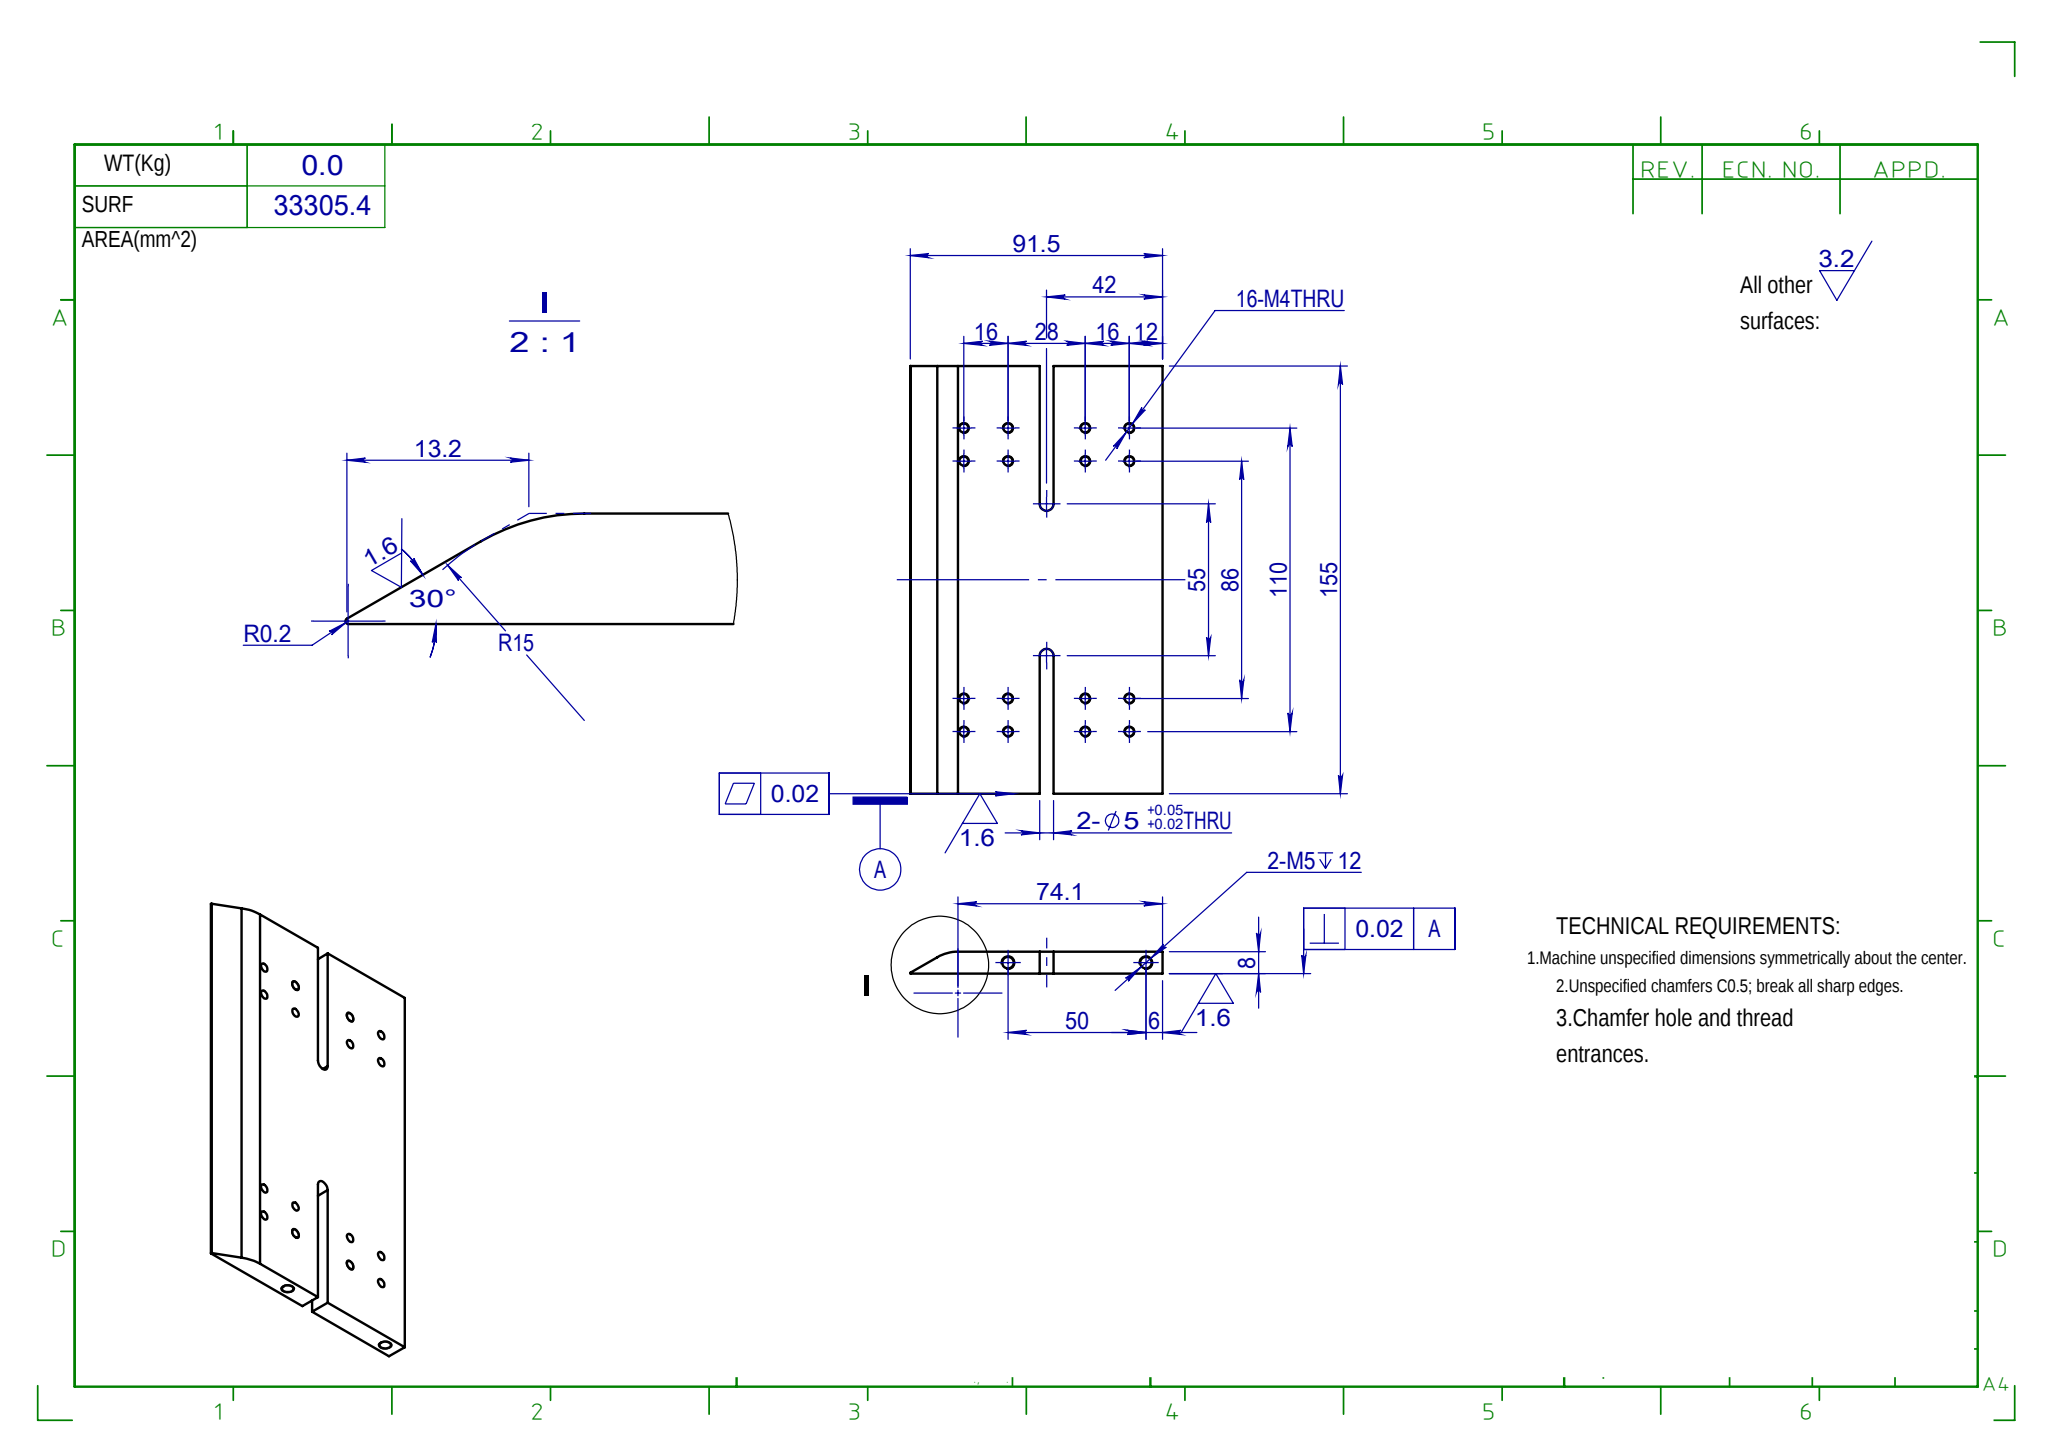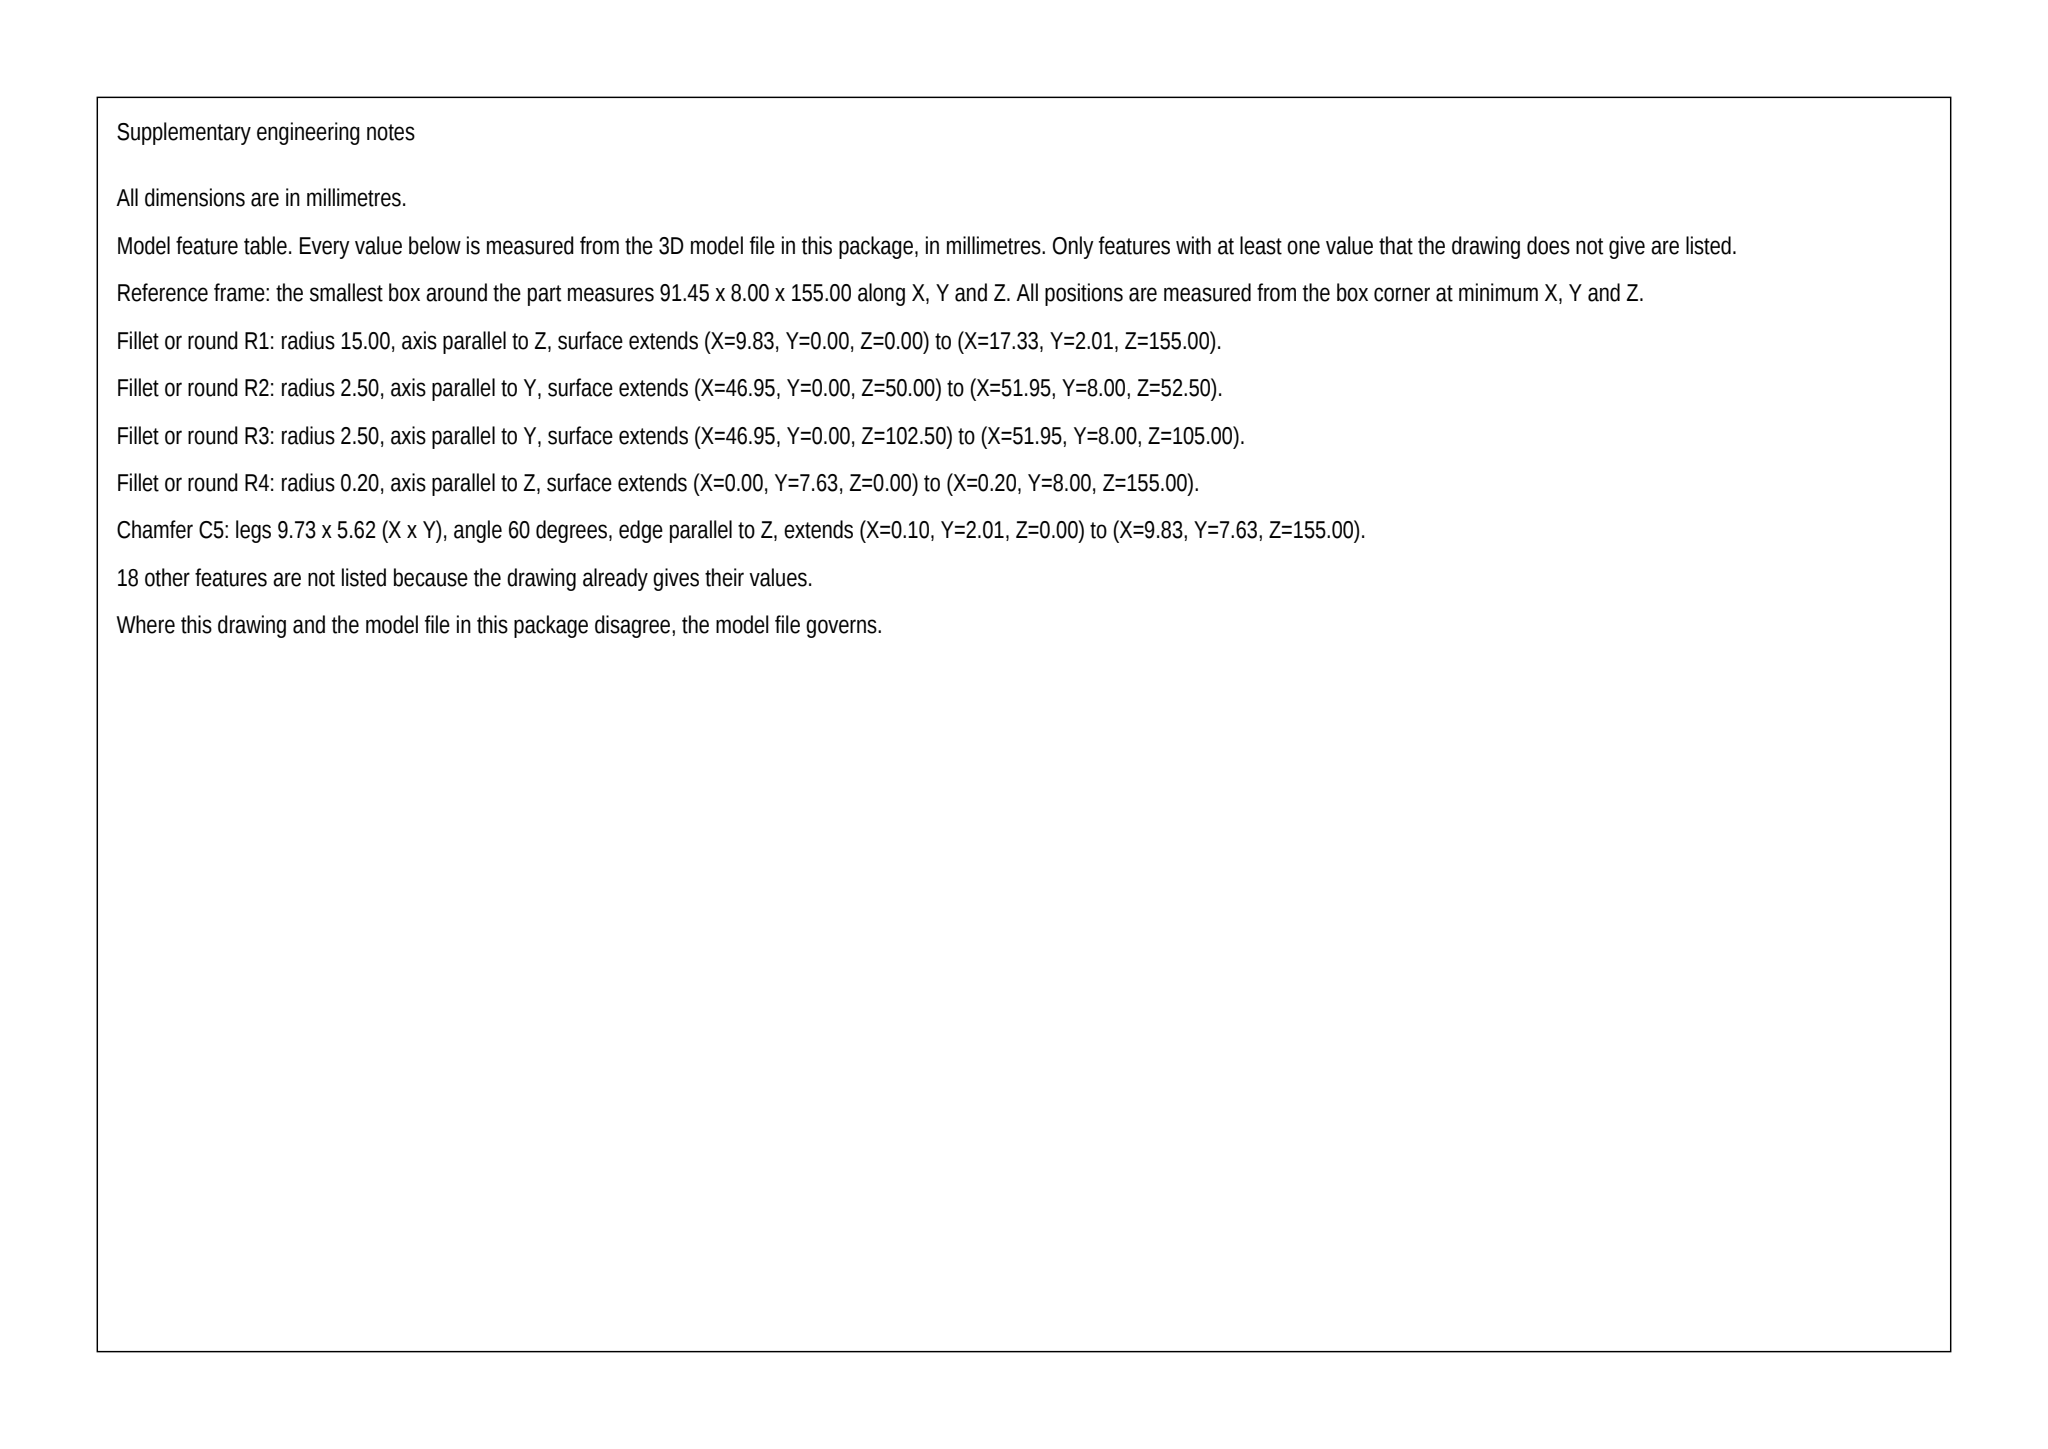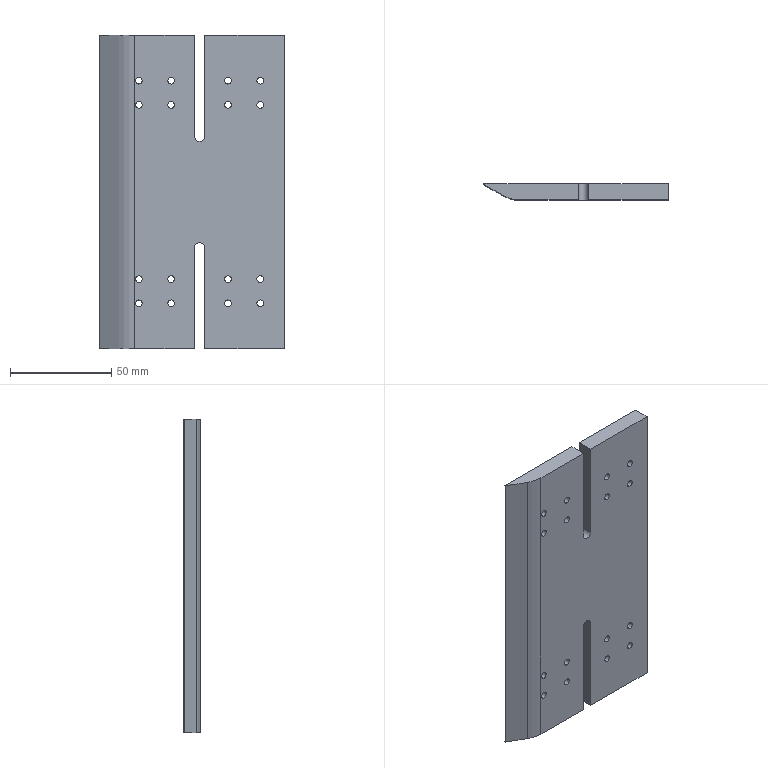Part | SolidWorks | mm | 1 solid | 58 faces | box 91.45 x 8 x 155 mm | volume 99608 mm3 | cylinder 42 | plane 12 | cone 4 | commonest cylinder face diameters 3.3 x32 4.2 x4 5 x3 0.4 x2 30 x1
build123d program:
from build123d import *

# Parameters (mm, degrees)
EXTRUDE1_DEPTH         = 155
FILLET1_R              = 0.2
M4_TAPPED_HOLE_2_D     = 3.3
M4_TAPPED_HOLE_2_DEPTH = 11.5
M4_TAPPED_HOLE_2_TIP   = 0.9914
CUT_EXTRUDE4_DEPTH     = 184.265
M4_TAPPED_HOLE_1_D     = 3.3
M5_TAPPED_HOLE_2_D     = 4.2
M5_TAPPED_HOLE_2_DEPTH = 14
M5_TAPPED_HOLE_2_TIP   = 1.262
SKETCH33_W             = 6
SKETCH33_H             = 155
CUT_EXTRUDE5_DEPTH     = 184.265
M4_TAPPED_HOLE_3_D     = 3.3


with BuildPart() as part:
    # Sketch1 → Extrude1 (new body)
    with BuildSketch(Plane.XY):
        with BuildLine():
            Line((-98, 8), (-87.624, 2.01))
            ThreePointArc((-87.624, 2.01), (-84.007, 0.5111), (-80.124, 0))
            Line((-80.124, 0), (0, 0))
            Line((0, 0), (0, 8))
            Line((0, 8), (-98, 8))
        make_face()
    extrude(amount=EXTRUDE1_DEPTH)

    # Fillet1
    fillet1_edges = [part.edges().sort_by_distance(p)[0] for p in [
        (-98, 8, 77.5),
    ]]
    fillet(fillet1_edges, radius=FILLET1_R)

    # M4 Tapped Hole 2
    with Locations(Plane(origin=(0, 8, 0), x_dir=(-1, 0, 0), z_dir=(0, 1, 0))):
        with Locations((78, 22.5), (18, 22.5), (78, 132.5), (18, 132.5)):
            Hole(M4_TAPPED_HOLE_2_D / 2, depth=M4_TAPPED_HOLE_2_DEPTH)
            with Locations((0, 0, -(M4_TAPPED_HOLE_2_DEPTH + M4_TAPPED_HOLE_2_TIP / 2))):  # 118° drill point
                Cone(0, M4_TAPPED_HOLE_2_D / 2, M4_TAPPED_HOLE_2_TIP, mode=Mode.SUBTRACT)

    # Sketch25 → Cut-Extrude4 (cut, through all)
    with BuildSketch(Plane(origin=(0, 8, 0), x_dir=(1, 0, 0), z_dir=(0, 1, 0))):
        with BuildLine():
            Line((-50.5, -50), (-50.5, 10))
            ThreePointArc((-50.5, 10), (-48, 12.5), (-45.5, 10))
            Line((-45.5, 10), (-45.5, -50))
            ThreePointArc((-45.5, -50), (-48, -52.5), (-50.5, -50))
        make_face()
        with BuildLine():
            Line((-50.5, -105), (-50.5, -165))
            ThreePointArc((-50.5, -165), (-48, -167.5), (-45.5, -165))
            Line((-45.5, -165), (-45.5, -105))
            ThreePointArc((-45.5, -105), (-48, -102.5), (-50.5, -105))
        make_face()
    extrude(amount=-CUT_EXTRUDE4_DEPTH, mode=Mode.SUBTRACT)

    # M4 Tapped Hole 1 (through all)
    with Locations(Plane.XZ):
        with Locations((-34, 132.5), (-34, 22.5), (-62, 132.5), (-62, 22.5)):
            Hole(M4_TAPPED_HOLE_1_D / 2)

    # M5 Tapped Hole 2
    with Locations(Plane(origin=(0, 0, 0), x_dir=(-1, 0, 0), z_dir=(0, 0, -1))):
        with Locations((12, 4), (62, 4)):
            Hole(M5_TAPPED_HOLE_2_D / 2, depth=M5_TAPPED_HOLE_2_DEPTH)
            with Locations((0, 0, -(M5_TAPPED_HOLE_2_DEPTH + M5_TAPPED_HOLE_2_TIP / 2))):  # 118° drill point
                Cone(0, M5_TAPPED_HOLE_2_D / 2, M5_TAPPED_HOLE_2_TIP, mode=Mode.SUBTRACT)

    # Sketch33 → Cut-Extrude5 (cut, through all)
    with BuildSketch(Plane(origin=(0, 8, 0), x_dir=(1, 0, 0), z_dir=(0, 1, 0))):
        with Locations((-3, -77.5)):
            Rectangle(SKETCH33_W, SKETCH33_H)
    extrude(amount=-CUT_EXTRUDE5_DEPTH, mode=Mode.SUBTRACT)

    # M4 Tapped Hole 3 (through all)
    with Locations(Plane(origin=(0, 8, 0), x_dir=(1, 0, 0), z_dir=(0, 1, 0))):
        with Locations((-78, -34.5), (-62, -34.5), (-34, -34.5), (-18, -34.5), (-78, -120.5), (-62, -120.5), (-34, -120.5), (-18, -120.5)):
            Hole(M4_TAPPED_HOLE_3_D / 2)


solid = part.part